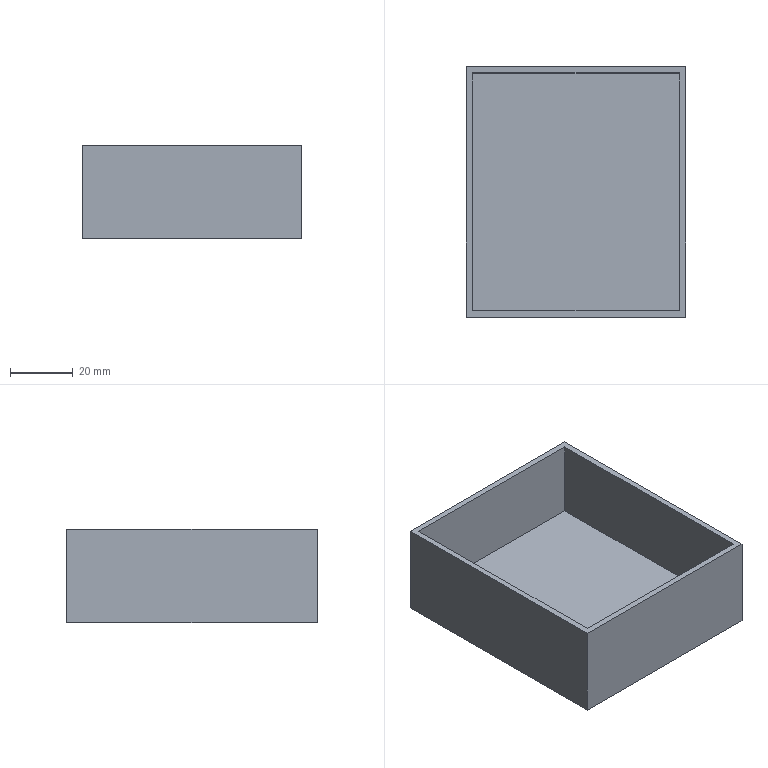Component | NX | REMOVABLE_STORAGE_1 | 1 solid | 11 faces | box 70 x 80 x 30 mm | volume 42600 mm3 | plane 11
STEP:
#1=CARTESIAN_POINT('',(0.,0.,0.));
#2=DIRECTION('',(0.,0.,1.));
#3=DIRECTION('',(1.,0.,0.));
#4=AXIS2_PLACEMENT_3D('',#1,#2,#3);
#5=CARTESIAN_POINT('',(145.,12.,35.));
#6=VERTEX_POINT('',#5);
#7=CARTESIAN_POINT('',(211.,12.,35.));
#8=VERTEX_POINT('',#7);
#9=CARTESIAN_POINT('',(145.,12.,35.));
#10=DIRECTION('',(1.,0.,0.));
#11=VECTOR('',#10,1.);
#12=LINE('',#9,#11);
#13=CARTESIAN_POINT('',(145.,12.,60.));
#14=DIRECTION('',(-0.,1.,0.));
#15=DIRECTION('',(-1.,-0.,0.));
#16=AXIS2_PLACEMENT_3D('',#13,#14,#15);
#17=PLANE('',#16);
#18=CARTESIAN_POINT('',(0.,-25.));
#19=DIRECTION('',(-1.,0.));
#20=VECTOR('',#19,1.);
#21=LINE('',#18,#20);
#22=(GEOMETRIC_REPRESENTATION_CONTEXT(2)PARAMETRIC_REPRESENTATION_CONTEXT()REPRESENTATION_CONTEXT('',''));
#23=DEFINITIONAL_REPRESENTATION('',(#21),#22);
#24=PCURVE('',#17,#23);
#25=CARTESIAN_POINT('',(143.,10.,35.));
#26=DIRECTION('',(0.,0.,1.));
#27=DIRECTION('',(1.,0.,0.));
#28=AXIS2_PLACEMENT_3D('',#25,#26,#27);
#29=PLANE('',#28);
#30=CARTESIAN_POINT('',(2.,2.));
#31=DIRECTION('',(1.,0.));
#32=VECTOR('',#31,1.);
#33=LINE('',#30,#32);
#34=(GEOMETRIC_REPRESENTATION_CONTEXT(2)PARAMETRIC_REPRESENTATION_CONTEXT()REPRESENTATION_CONTEXT('',''));
#35=DEFINITIONAL_REPRESENTATION('',(#33),#34);
#36=PCURVE('',#29,#35);
#37=SURFACE_CURVE('',#12,(#24,#36),.PCURVE_S1.);
#38=EDGE_CURVE('',#6,#8,#37,.T.);
#39=ORIENTED_EDGE('',*,*,#38,.F.);
#40=CARTESIAN_POINT('',(145.,12.,60.));
#41=VERTEX_POINT('',#40);
#42=CARTESIAN_POINT('',(145.,12.,60.));
#43=DIRECTION('',(0.,0.,-1.));
#44=VECTOR('',#43,1.);
#45=LINE('',#42,#44);
#46=CARTESIAN_POINT('',(0.,0.));
#47=DIRECTION('',(0.,-1.));
#48=VECTOR('',#47,1.);
#49=LINE('',#46,#48);
#50=(GEOMETRIC_REPRESENTATION_CONTEXT(2)PARAMETRIC_REPRESENTATION_CONTEXT()REPRESENTATION_CONTEXT('',''));
#51=DEFINITIONAL_REPRESENTATION('',(#49),#50);
#52=PCURVE('',#17,#51);
#53=CARTESIAN_POINT('',(145.,88.,60.));
#54=DIRECTION('',(1.,0.,0.));
#55=DIRECTION('',(-0.,1.,0.));
#56=AXIS2_PLACEMENT_3D('',#53,#54,#55);
#57=PLANE('',#56);
#58=CARTESIAN_POINT('',(-76.,0.));
#59=DIRECTION('',(0.,-1.));
#60=VECTOR('',#59,1.);
#61=LINE('',#58,#60);
#62=(GEOMETRIC_REPRESENTATION_CONTEXT(2)PARAMETRIC_REPRESENTATION_CONTEXT()REPRESENTATION_CONTEXT('',''));
#63=DEFINITIONAL_REPRESENTATION('',(#61),#62);
#64=PCURVE('',#57,#63);
#65=SURFACE_CURVE('',#45,(#52,#64),.PCURVE_S1.);
#66=EDGE_CURVE('',#41,#6,#65,.T.);
#67=ORIENTED_EDGE('',*,*,#66,.F.);
#68=CARTESIAN_POINT('',(211.,12.,60.));
#69=VERTEX_POINT('',#68);
#70=CARTESIAN_POINT('',(145.,12.,60.));
#71=DIRECTION('',(1.,0.,0.));
#72=VECTOR('',#71,1.);
#73=LINE('',#70,#72);
#74=CARTESIAN_POINT('',(0.,0.));
#75=DIRECTION('',(-1.,0.));
#76=VECTOR('',#75,1.);
#77=LINE('',#74,#76);
#78=(GEOMETRIC_REPRESENTATION_CONTEXT(2)PARAMETRIC_REPRESENTATION_CONTEXT()REPRESENTATION_CONTEXT('',''));
#79=DEFINITIONAL_REPRESENTATION('',(#77),#78);
#80=PCURVE('',#17,#79);
#81=CARTESIAN_POINT('',(143.,10.,60.));
#82=DIRECTION('',(0.,0.,-1.));
#83=DIRECTION('',(-1.,0.,0.));
#84=AXIS2_PLACEMENT_3D('',#81,#82,#83);
#85=PLANE('',#84);
#86=CARTESIAN_POINT('',(-2.,2.));
#87=DIRECTION('',(-1.,0.));
#88=VECTOR('',#87,1.);
#89=LINE('',#86,#88);
#90=(GEOMETRIC_REPRESENTATION_CONTEXT(2)PARAMETRIC_REPRESENTATION_CONTEXT()REPRESENTATION_CONTEXT('',''));
#91=DEFINITIONAL_REPRESENTATION('',(#89),#90);
#92=PCURVE('',#85,#91);
#93=SURFACE_CURVE('',#73,(#80,#92),.PCURVE_S1.);
#94=EDGE_CURVE('',#41,#69,#93,.T.);
#95=ORIENTED_EDGE('',*,*,#94,.T.);
#96=CARTESIAN_POINT('',(211.,12.,60.));
#97=DIRECTION('',(0.,0.,-1.));
#98=VECTOR('',#97,1.);
#99=LINE('',#96,#98);
#100=CARTESIAN_POINT('',(-66.,0.));
#101=DIRECTION('',(0.,-1.));
#102=VECTOR('',#101,1.);
#103=LINE('',#100,#102);
#104=(GEOMETRIC_REPRESENTATION_CONTEXT(2)PARAMETRIC_REPRESENTATION_CONTEXT()REPRESENTATION_CONTEXT('',''));
#105=DEFINITIONAL_REPRESENTATION('',(#103),#104);
#106=PCURVE('',#17,#105);
#107=CARTESIAN_POINT('',(211.,12.,60.));
#108=DIRECTION('',(-1.,0.,0.));
#109=DIRECTION('',(-0.,-1.,0.));
#110=AXIS2_PLACEMENT_3D('',#107,#108,#109);
#111=PLANE('',#110);
#112=CARTESIAN_POINT('',(0.,0.));
#113=DIRECTION('',(0.,-1.));
#114=VECTOR('',#113,1.);
#115=LINE('',#112,#114);
#116=(GEOMETRIC_REPRESENTATION_CONTEXT(2)PARAMETRIC_REPRESENTATION_CONTEXT()REPRESENTATION_CONTEXT('',''));
#117=DEFINITIONAL_REPRESENTATION('',(#115),#116);
#118=PCURVE('',#111,#117);
#119=SURFACE_CURVE('',#99,(#106,#118),.PCURVE_S1.);
#120=EDGE_CURVE('',#69,#8,#119,.T.);
#121=ORIENTED_EDGE('',*,*,#120,.T.);
#122=EDGE_LOOP('',(#39,#67,#95,#121));
#123=FACE_BOUND('',#122,.T.);
#124=ADVANCED_FACE('',(#123),#17,.T.);
#125=CARTESIAN_POINT('',(211.,88.,35.));
#126=VERTEX_POINT('',#125);
#127=CARTESIAN_POINT('',(211.,12.,35.));
#128=DIRECTION('',(0.,1.,0.));
#129=VECTOR('',#128,1.);
#130=LINE('',#127,#129);
#131=CARTESIAN_POINT('',(0.,-25.));
#132=DIRECTION('',(-1.,0.));
#133=VECTOR('',#132,1.);
#134=LINE('',#131,#133);
#135=(GEOMETRIC_REPRESENTATION_CONTEXT(2)PARAMETRIC_REPRESENTATION_CONTEXT()REPRESENTATION_CONTEXT('',''));
#136=DEFINITIONAL_REPRESENTATION('',(#134),#135);
#137=PCURVE('',#111,#136);
#138=CARTESIAN_POINT('',(68.,2.));
#139=DIRECTION('',(0.,1.));
#140=VECTOR('',#139,1.);
#141=LINE('',#138,#140);
#142=(GEOMETRIC_REPRESENTATION_CONTEXT(2)PARAMETRIC_REPRESENTATION_CONTEXT()REPRESENTATION_CONTEXT('',''));
#143=DEFINITIONAL_REPRESENTATION('',(#141),#142);
#144=PCURVE('',#29,#143);
#145=SURFACE_CURVE('',#130,(#137,#144),.PCURVE_S1.);
#146=EDGE_CURVE('',#8,#126,#145,.T.);
#147=ORIENTED_EDGE('',*,*,#146,.F.);
#148=ORIENTED_EDGE('',*,*,#120,.F.);
#149=CARTESIAN_POINT('',(211.,88.,60.));
#150=VERTEX_POINT('',#149);
#151=CARTESIAN_POINT('',(211.,12.,60.));
#152=DIRECTION('',(0.,1.,0.));
#153=VECTOR('',#152,1.);
#154=LINE('',#151,#153);
#155=CARTESIAN_POINT('',(0.,0.));
#156=DIRECTION('',(-1.,0.));
#157=VECTOR('',#156,1.);
#158=LINE('',#155,#157);
#159=(GEOMETRIC_REPRESENTATION_CONTEXT(2)PARAMETRIC_REPRESENTATION_CONTEXT()REPRESENTATION_CONTEXT('',''));
#160=DEFINITIONAL_REPRESENTATION('',(#158),#159);
#161=PCURVE('',#111,#160);
#162=CARTESIAN_POINT('',(-68.,2.));
#163=DIRECTION('',(-0.,1.));
#164=VECTOR('',#163,1.);
#165=LINE('',#162,#164);
#166=(GEOMETRIC_REPRESENTATION_CONTEXT(2)PARAMETRIC_REPRESENTATION_CONTEXT()REPRESENTATION_CONTEXT('',''));
#167=DEFINITIONAL_REPRESENTATION('',(#165),#166);
#168=PCURVE('',#85,#167);
#169=SURFACE_CURVE('',#154,(#161,#168),.PCURVE_S1.);
#170=EDGE_CURVE('',#69,#150,#169,.T.);
#171=ORIENTED_EDGE('',*,*,#170,.T.);
#172=CARTESIAN_POINT('',(211.,88.,60.));
#173=DIRECTION('',(0.,0.,-1.));
#174=VECTOR('',#173,1.);
#175=LINE('',#172,#174);
#176=CARTESIAN_POINT('',(-76.,0.));
#177=DIRECTION('',(0.,-1.));
#178=VECTOR('',#177,1.);
#179=LINE('',#176,#178);
#180=(GEOMETRIC_REPRESENTATION_CONTEXT(2)PARAMETRIC_REPRESENTATION_CONTEXT()REPRESENTATION_CONTEXT('',''));
#181=DEFINITIONAL_REPRESENTATION('',(#179),#180);
#182=PCURVE('',#111,#181);
#183=CARTESIAN_POINT('',(211.,88.,60.));
#184=DIRECTION('',(-0.,-1.,0.));
#185=DIRECTION('',(1.,-0.,0.));
#186=AXIS2_PLACEMENT_3D('',#183,#184,#185);
#187=PLANE('',#186);
#188=CARTESIAN_POINT('',(0.,0.));
#189=DIRECTION('',(0.,-1.));
#190=VECTOR('',#189,1.);
#191=LINE('',#188,#190);
#192=(GEOMETRIC_REPRESENTATION_CONTEXT(2)PARAMETRIC_REPRESENTATION_CONTEXT()REPRESENTATION_CONTEXT('',''));
#193=DEFINITIONAL_REPRESENTATION('',(#191),#192);
#194=PCURVE('',#187,#193);
#195=SURFACE_CURVE('',#175,(#182,#194),.PCURVE_S1.);
#196=EDGE_CURVE('',#150,#126,#195,.T.);
#197=ORIENTED_EDGE('',*,*,#196,.T.);
#198=EDGE_LOOP('',(#147,#148,#171,#197));
#199=FACE_BOUND('',#198,.T.);
#200=ADVANCED_FACE('',(#199),#111,.T.);
#201=CARTESIAN_POINT('',(145.,88.,35.));
#202=VERTEX_POINT('',#201);
#203=CARTESIAN_POINT('',(211.,88.,35.));
#204=DIRECTION('',(-1.,0.,0.));
#205=VECTOR('',#204,1.);
#206=LINE('',#203,#205);
#207=CARTESIAN_POINT('',(0.,-25.));
#208=DIRECTION('',(-1.,0.));
#209=VECTOR('',#208,1.);
#210=LINE('',#207,#209);
#211=(GEOMETRIC_REPRESENTATION_CONTEXT(2)PARAMETRIC_REPRESENTATION_CONTEXT()REPRESENTATION_CONTEXT('',''));
#212=DEFINITIONAL_REPRESENTATION('',(#210),#211);
#213=PCURVE('',#187,#212);
#214=CARTESIAN_POINT('',(68.,78.));
#215=DIRECTION('',(-1.,0.));
#216=VECTOR('',#215,1.);
#217=LINE('',#214,#216);
#218=(GEOMETRIC_REPRESENTATION_CONTEXT(2)PARAMETRIC_REPRESENTATION_CONTEXT()REPRESENTATION_CONTEXT('',''));
#219=DEFINITIONAL_REPRESENTATION('',(#217),#218);
#220=PCURVE('',#29,#219);
#221=SURFACE_CURVE('',#206,(#213,#220),.PCURVE_S1.);
#222=EDGE_CURVE('',#126,#202,#221,.T.);
#223=ORIENTED_EDGE('',*,*,#222,.F.);
#224=ORIENTED_EDGE('',*,*,#196,.F.);
#225=CARTESIAN_POINT('',(145.,88.,60.));
#226=VERTEX_POINT('',#225);
#227=CARTESIAN_POINT('',(211.,88.,60.));
#228=DIRECTION('',(-1.,0.,0.));
#229=VECTOR('',#228,1.);
#230=LINE('',#227,#229);
#231=CARTESIAN_POINT('',(0.,0.));
#232=DIRECTION('',(-1.,0.));
#233=VECTOR('',#232,1.);
#234=LINE('',#231,#233);
#235=(GEOMETRIC_REPRESENTATION_CONTEXT(2)PARAMETRIC_REPRESENTATION_CONTEXT()REPRESENTATION_CONTEXT('',''));
#236=DEFINITIONAL_REPRESENTATION('',(#234),#235);
#237=PCURVE('',#187,#236);
#238=CARTESIAN_POINT('',(-68.,78.));
#239=DIRECTION('',(1.,0.));
#240=VECTOR('',#239,1.);
#241=LINE('',#238,#240);
#242=(GEOMETRIC_REPRESENTATION_CONTEXT(2)PARAMETRIC_REPRESENTATION_CONTEXT()REPRESENTATION_CONTEXT('',''));
#243=DEFINITIONAL_REPRESENTATION('',(#241),#242);
#244=PCURVE('',#85,#243);
#245=SURFACE_CURVE('',#230,(#237,#244),.PCURVE_S1.);
#246=EDGE_CURVE('',#150,#226,#245,.T.);
#247=ORIENTED_EDGE('',*,*,#246,.T.);
#248=CARTESIAN_POINT('',(145.,88.,60.));
#249=DIRECTION('',(0.,0.,-1.));
#250=VECTOR('',#249,1.);
#251=LINE('',#248,#250);
#252=CARTESIAN_POINT('',(-66.,0.));
#253=DIRECTION('',(0.,-1.));
#254=VECTOR('',#253,1.);
#255=LINE('',#252,#254);
#256=(GEOMETRIC_REPRESENTATION_CONTEXT(2)PARAMETRIC_REPRESENTATION_CONTEXT()REPRESENTATION_CONTEXT('',''));
#257=DEFINITIONAL_REPRESENTATION('',(#255),#256);
#258=PCURVE('',#187,#257);
#259=CARTESIAN_POINT('',(0.,0.));
#260=DIRECTION('',(0.,-1.));
#261=VECTOR('',#260,1.);
#262=LINE('',#259,#261);
#263=(GEOMETRIC_REPRESENTATION_CONTEXT(2)PARAMETRIC_REPRESENTATION_CONTEXT()REPRESENTATION_CONTEXT('',''));
#264=DEFINITIONAL_REPRESENTATION('',(#262),#263);
#265=PCURVE('',#57,#264);
#266=SURFACE_CURVE('',#251,(#258,#265),.PCURVE_S1.);
#267=EDGE_CURVE('',#226,#202,#266,.T.);
#268=ORIENTED_EDGE('',*,*,#267,.T.);
#269=EDGE_LOOP('',(#223,#224,#247,#268));
#270=FACE_BOUND('',#269,.T.);
#271=ADVANCED_FACE('',(#270),#187,.T.);
#272=CARTESIAN_POINT('',(143.,90.,30.));
#273=VERTEX_POINT('',#272);
#274=CARTESIAN_POINT('',(213.,90.,30.));
#275=VERTEX_POINT('',#274);
#276=CARTESIAN_POINT('',(143.,90.,30.));
#277=DIRECTION('',(1.,0.,0.));
#278=VECTOR('',#277,1.);
#279=LINE('',#276,#278);
#280=CARTESIAN_POINT('',(143.,90.,60.));
#281=DIRECTION('',(0.,1.,0.));
#282=DIRECTION('',(0.,0.,1.));
#283=AXIS2_PLACEMENT_3D('',#280,#281,#282);
#284=PLANE('',#283);
#285=CARTESIAN_POINT('',(-30.,0.));
#286=DIRECTION('',(0.,1.));
#287=VECTOR('',#286,1.);
#288=LINE('',#285,#287);
#289=(GEOMETRIC_REPRESENTATION_CONTEXT(2)PARAMETRIC_REPRESENTATION_CONTEXT()REPRESENTATION_CONTEXT('',''));
#290=DEFINITIONAL_REPRESENTATION('',(#288),#289);
#291=PCURVE('',#284,#290);
#292=CARTESIAN_POINT('',(143.,10.,30.));
#293=DIRECTION('',(0.,0.,-1.));
#294=DIRECTION('',(-1.,0.,0.));
#295=AXIS2_PLACEMENT_3D('',#292,#293,#294);
#296=PLANE('',#295);
#297=CARTESIAN_POINT('',(0.,80.));
#298=DIRECTION('',(-1.,0.));
#299=VECTOR('',#298,1.);
#300=LINE('',#297,#299);
#301=(GEOMETRIC_REPRESENTATION_CONTEXT(2)PARAMETRIC_REPRESENTATION_CONTEXT()REPRESENTATION_CONTEXT('',''));
#302=DEFINITIONAL_REPRESENTATION('',(#300),#301);
#303=PCURVE('',#296,#302);
#304=SURFACE_CURVE('',#279,(#291,#303),.PCURVE_S1.);
#305=EDGE_CURVE('',#273,#275,#304,.T.);
#306=ORIENTED_EDGE('',*,*,#305,.F.);
#307=CARTESIAN_POINT('',(143.,90.,60.));
#308=VERTEX_POINT('',#307);
#309=CARTESIAN_POINT('',(143.,90.,60.));
#310=DIRECTION('',(0.,0.,-1.));
#311=VECTOR('',#310,1.);
#312=LINE('',#309,#311);
#313=CARTESIAN_POINT('',(0.,0.));
#314=DIRECTION('',(-1.,0.));
#315=VECTOR('',#314,1.);
#316=LINE('',#313,#315);
#317=(GEOMETRIC_REPRESENTATION_CONTEXT(2)PARAMETRIC_REPRESENTATION_CONTEXT()REPRESENTATION_CONTEXT('',''));
#318=DEFINITIONAL_REPRESENTATION('',(#316),#317);
#319=PCURVE('',#284,#318);
#320=CARTESIAN_POINT('',(143.,10.,60.));
#321=DIRECTION('',(-1.,0.,0.));
#322=DIRECTION('',(0.,0.,1.));
#323=AXIS2_PLACEMENT_3D('',#320,#321,#322);
#324=PLANE('',#323);
#325=CARTESIAN_POINT('',(0.,80.));
#326=DIRECTION('',(-1.,0.));
#327=VECTOR('',#326,1.);
#328=LINE('',#325,#327);
#329=(GEOMETRIC_REPRESENTATION_CONTEXT(2)PARAMETRIC_REPRESENTATION_CONTEXT()REPRESENTATION_CONTEXT('',''));
#330=DEFINITIONAL_REPRESENTATION('',(#328),#329);
#331=PCURVE('',#324,#330);
#332=SURFACE_CURVE('',#312,(#319,#331),.PCURVE_S1.);
#333=EDGE_CURVE('',#308,#273,#332,.T.);
#334=ORIENTED_EDGE('',*,*,#333,.F.);
#335=CARTESIAN_POINT('',(213.,90.,60.));
#336=VERTEX_POINT('',#335);
#337=CARTESIAN_POINT('',(143.,90.,60.));
#338=DIRECTION('',(1.,0.,0.));
#339=VECTOR('',#338,1.);
#340=LINE('',#337,#339);
#341=CARTESIAN_POINT('',(0.,0.));
#342=DIRECTION('',(0.,1.));
#343=VECTOR('',#342,1.);
#344=LINE('',#341,#343);
#345=(GEOMETRIC_REPRESENTATION_CONTEXT(2)PARAMETRIC_REPRESENTATION_CONTEXT()REPRESENTATION_CONTEXT('',''));
#346=DEFINITIONAL_REPRESENTATION('',(#344),#345);
#347=PCURVE('',#284,#346);
#348=CARTESIAN_POINT('',(0.,80.));
#349=DIRECTION('',(-1.,0.));
#350=VECTOR('',#349,1.);
#351=LINE('',#348,#350);
#352=(GEOMETRIC_REPRESENTATION_CONTEXT(2)PARAMETRIC_REPRESENTATION_CONTEXT()REPRESENTATION_CONTEXT('',''));
#353=DEFINITIONAL_REPRESENTATION('',(#351),#352);
#354=PCURVE('',#85,#353);
#355=SURFACE_CURVE('',#340,(#347,#354),.PCURVE_S1.);
#356=EDGE_CURVE('',#308,#336,#355,.T.);
#357=ORIENTED_EDGE('',*,*,#356,.T.);
#358=CARTESIAN_POINT('',(213.,90.,60.));
#359=DIRECTION('',(0.,0.,-1.));
#360=VECTOR('',#359,1.);
#361=LINE('',#358,#360);
#362=CARTESIAN_POINT('',(0.,70.));
#363=DIRECTION('',(-1.,0.));
#364=VECTOR('',#363,1.);
#365=LINE('',#362,#364);
#366=(GEOMETRIC_REPRESENTATION_CONTEXT(2)PARAMETRIC_REPRESENTATION_CONTEXT()REPRESENTATION_CONTEXT('',''));
#367=DEFINITIONAL_REPRESENTATION('',(#365),#366);
#368=PCURVE('',#284,#367);
#369=CARTESIAN_POINT('',(213.,90.,60.));
#370=DIRECTION('',(1.,0.,0.));
#371=DIRECTION('',(0.,0.,-1.));
#372=AXIS2_PLACEMENT_3D('',#369,#370,#371);
#373=PLANE('',#372);
#374=CARTESIAN_POINT('',(0.,0.));
#375=DIRECTION('',(1.,0.));
#376=VECTOR('',#375,1.);
#377=LINE('',#374,#376);
#378=(GEOMETRIC_REPRESENTATION_CONTEXT(2)PARAMETRIC_REPRESENTATION_CONTEXT()REPRESENTATION_CONTEXT('',''));
#379=DEFINITIONAL_REPRESENTATION('',(#377),#378);
#380=PCURVE('',#373,#379);
#381=SURFACE_CURVE('',#361,(#368,#380),.PCURVE_S1.);
#382=EDGE_CURVE('',#336,#275,#381,.T.);
#383=ORIENTED_EDGE('',*,*,#382,.T.);
#384=EDGE_LOOP('',(#306,#334,#357,#383));
#385=FACE_BOUND('',#384,.T.);
#386=ADVANCED_FACE('',(#385),#284,.T.);
#387=CARTESIAN_POINT('',(213.,10.,30.));
#388=VERTEX_POINT('',#387);
#389=CARTESIAN_POINT('',(213.,90.,30.));
#390=DIRECTION('',(0.,-1.,0.));
#391=VECTOR('',#390,1.);
#392=LINE('',#389,#391);
#393=CARTESIAN_POINT('',(30.,0.));
#394=DIRECTION('',(0.,-1.));
#395=VECTOR('',#394,1.);
#396=LINE('',#393,#395);
#397=(GEOMETRIC_REPRESENTATION_CONTEXT(2)PARAMETRIC_REPRESENTATION_CONTEXT()REPRESENTATION_CONTEXT('',''));
#398=DEFINITIONAL_REPRESENTATION('',(#396),#397);
#399=PCURVE('',#373,#398);
#400=CARTESIAN_POINT('',(-70.,80.));
#401=DIRECTION('',(0.,-1.));
#402=VECTOR('',#401,1.);
#403=LINE('',#400,#402);
#404=(GEOMETRIC_REPRESENTATION_CONTEXT(2)PARAMETRIC_REPRESENTATION_CONTEXT()REPRESENTATION_CONTEXT('',''));
#405=DEFINITIONAL_REPRESENTATION('',(#403),#404);
#406=PCURVE('',#296,#405);
#407=SURFACE_CURVE('',#392,(#399,#406),.PCURVE_S1.);
#408=EDGE_CURVE('',#275,#388,#407,.T.);
#409=ORIENTED_EDGE('',*,*,#408,.F.);
#410=ORIENTED_EDGE('',*,*,#382,.F.);
#411=CARTESIAN_POINT('',(213.,10.,60.));
#412=VERTEX_POINT('',#411);
#413=CARTESIAN_POINT('',(213.,90.,60.));
#414=DIRECTION('',(0.,-1.,0.));
#415=VECTOR('',#414,1.);
#416=LINE('',#413,#415);
#417=CARTESIAN_POINT('',(0.,0.));
#418=DIRECTION('',(0.,-1.));
#419=VECTOR('',#418,1.);
#420=LINE('',#417,#419);
#421=(GEOMETRIC_REPRESENTATION_CONTEXT(2)PARAMETRIC_REPRESENTATION_CONTEXT()REPRESENTATION_CONTEXT('',''));
#422=DEFINITIONAL_REPRESENTATION('',(#420),#421);
#423=PCURVE('',#373,#422);
#424=CARTESIAN_POINT('',(-70.,80.));
#425=DIRECTION('',(0.,-1.));
#426=VECTOR('',#425,1.);
#427=LINE('',#424,#426);
#428=(GEOMETRIC_REPRESENTATION_CONTEXT(2)PARAMETRIC_REPRESENTATION_CONTEXT()REPRESENTATION_CONTEXT('',''));
#429=DEFINITIONAL_REPRESENTATION('',(#427),#428);
#430=PCURVE('',#85,#429);
#431=SURFACE_CURVE('',#416,(#423,#430),.PCURVE_S1.);
#432=EDGE_CURVE('',#336,#412,#431,.T.);
#433=ORIENTED_EDGE('',*,*,#432,.T.);
#434=CARTESIAN_POINT('',(213.,10.,60.));
#435=DIRECTION('',(0.,0.,-1.));
#436=VECTOR('',#435,1.);
#437=LINE('',#434,#436);
#438=CARTESIAN_POINT('',(0.,-80.));
#439=DIRECTION('',(1.,0.));
#440=VECTOR('',#439,1.);
#441=LINE('',#438,#440);
#442=(GEOMETRIC_REPRESENTATION_CONTEXT(2)PARAMETRIC_REPRESENTATION_CONTEXT()REPRESENTATION_CONTEXT('',''));
#443=DEFINITIONAL_REPRESENTATION('',(#441),#442);
#444=PCURVE('',#373,#443);
#445=CARTESIAN_POINT('',(213.,10.,60.));
#446=DIRECTION('',(0.,-1.,0.));
#447=DIRECTION('',(0.,0.,-1.));
#448=AXIS2_PLACEMENT_3D('',#445,#446,#447);
#449=PLANE('',#448);
#450=CARTESIAN_POINT('',(0.,0.));
#451=DIRECTION('',(1.,0.));
#452=VECTOR('',#451,1.);
#453=LINE('',#450,#452);
#454=(GEOMETRIC_REPRESENTATION_CONTEXT(2)PARAMETRIC_REPRESENTATION_CONTEXT()REPRESENTATION_CONTEXT('',''));
#455=DEFINITIONAL_REPRESENTATION('',(#453),#454);
#456=PCURVE('',#449,#455);
#457=SURFACE_CURVE('',#437,(#444,#456),.PCURVE_S1.);
#458=EDGE_CURVE('',#412,#388,#457,.T.);
#459=ORIENTED_EDGE('',*,*,#458,.T.);
#460=EDGE_LOOP('',(#409,#410,#433,#459));
#461=FACE_BOUND('',#460,.T.);
#462=ADVANCED_FACE('',(#461),#373,.T.);
#463=CARTESIAN_POINT('',(143.,10.,30.));
#464=VERTEX_POINT('',#463);
#465=CARTESIAN_POINT('',(213.,10.,30.));
#466=DIRECTION('',(-1.,0.,0.));
#467=VECTOR('',#466,1.);
#468=LINE('',#465,#467);
#469=CARTESIAN_POINT('',(30.,0.));
#470=DIRECTION('',(0.,-1.));
#471=VECTOR('',#470,1.);
#472=LINE('',#469,#471);
#473=(GEOMETRIC_REPRESENTATION_CONTEXT(2)PARAMETRIC_REPRESENTATION_CONTEXT()REPRESENTATION_CONTEXT('',''));
#474=DEFINITIONAL_REPRESENTATION('',(#472),#473);
#475=PCURVE('',#449,#474);
#476=CARTESIAN_POINT('',(-70.,0.));
#477=DIRECTION('',(1.,0.));
#478=VECTOR('',#477,1.);
#479=LINE('',#476,#478);
#480=(GEOMETRIC_REPRESENTATION_CONTEXT(2)PARAMETRIC_REPRESENTATION_CONTEXT()REPRESENTATION_CONTEXT('',''));
#481=DEFINITIONAL_REPRESENTATION('',(#479),#480);
#482=PCURVE('',#296,#481);
#483=SURFACE_CURVE('',#468,(#475,#482),.PCURVE_S1.);
#484=EDGE_CURVE('',#388,#464,#483,.T.);
#485=ORIENTED_EDGE('',*,*,#484,.F.);
#486=ORIENTED_EDGE('',*,*,#458,.F.);
#487=CARTESIAN_POINT('',(143.,10.,60.));
#488=VERTEX_POINT('',#487);
#489=CARTESIAN_POINT('',(213.,10.,60.));
#490=DIRECTION('',(-1.,0.,0.));
#491=VECTOR('',#490,1.);
#492=LINE('',#489,#491);
#493=CARTESIAN_POINT('',(0.,0.));
#494=DIRECTION('',(0.,-1.));
#495=VECTOR('',#494,1.);
#496=LINE('',#493,#495);
#497=(GEOMETRIC_REPRESENTATION_CONTEXT(2)PARAMETRIC_REPRESENTATION_CONTEXT()REPRESENTATION_CONTEXT('',''));
#498=DEFINITIONAL_REPRESENTATION('',(#496),#497);
#499=PCURVE('',#449,#498);
#500=CARTESIAN_POINT('',(-70.,0.));
#501=DIRECTION('',(1.,0.));
#502=VECTOR('',#501,1.);
#503=LINE('',#500,#502);
#504=(GEOMETRIC_REPRESENTATION_CONTEXT(2)PARAMETRIC_REPRESENTATION_CONTEXT()REPRESENTATION_CONTEXT('',''));
#505=DEFINITIONAL_REPRESENTATION('',(#503),#504);
#506=PCURVE('',#85,#505);
#507=SURFACE_CURVE('',#492,(#499,#506),.PCURVE_S1.);
#508=EDGE_CURVE('',#412,#488,#507,.T.);
#509=ORIENTED_EDGE('',*,*,#508,.T.);
#510=CARTESIAN_POINT('',(143.,10.,60.));
#511=DIRECTION('',(0.,0.,-1.));
#512=VECTOR('',#511,1.);
#513=LINE('',#510,#512);
#514=CARTESIAN_POINT('',(0.,-70.));
#515=DIRECTION('',(1.,0.));
#516=VECTOR('',#515,1.);
#517=LINE('',#514,#516);
#518=(GEOMETRIC_REPRESENTATION_CONTEXT(2)PARAMETRIC_REPRESENTATION_CONTEXT()REPRESENTATION_CONTEXT('',''));
#519=DEFINITIONAL_REPRESENTATION('',(#517),#518);
#520=PCURVE('',#449,#519);
#521=CARTESIAN_POINT('',(0.,0.));
#522=DIRECTION('',(-1.,0.));
#523=VECTOR('',#522,1.);
#524=LINE('',#521,#523);
#525=(GEOMETRIC_REPRESENTATION_CONTEXT(2)PARAMETRIC_REPRESENTATION_CONTEXT()REPRESENTATION_CONTEXT('',''));
#526=DEFINITIONAL_REPRESENTATION('',(#524),#525);
#527=PCURVE('',#324,#526);
#528=SURFACE_CURVE('',#513,(#520,#527),.PCURVE_S1.);
#529=EDGE_CURVE('',#488,#464,#528,.T.);
#530=ORIENTED_EDGE('',*,*,#529,.T.);
#531=EDGE_LOOP('',(#485,#486,#509,#530));
#532=FACE_BOUND('',#531,.T.);
#533=ADVANCED_FACE('',(#532),#449,.T.);
#534=CARTESIAN_POINT('',(143.,10.,30.));
#535=DIRECTION('',(0.,1.,0.));
#536=VECTOR('',#535,1.);
#537=LINE('',#534,#536);
#538=CARTESIAN_POINT('',(-30.,0.));
#539=DIRECTION('',(0.,1.));
#540=VECTOR('',#539,1.);
#541=LINE('',#538,#540);
#542=(GEOMETRIC_REPRESENTATION_CONTEXT(2)PARAMETRIC_REPRESENTATION_CONTEXT()REPRESENTATION_CONTEXT('',''));
#543=DEFINITIONAL_REPRESENTATION('',(#541),#542);
#544=PCURVE('',#324,#543);
#545=CARTESIAN_POINT('',(0.,0.));
#546=DIRECTION('',(0.,1.));
#547=VECTOR('',#546,1.);
#548=LINE('',#545,#547);
#549=(GEOMETRIC_REPRESENTATION_CONTEXT(2)PARAMETRIC_REPRESENTATION_CONTEXT()REPRESENTATION_CONTEXT('',''));
#550=DEFINITIONAL_REPRESENTATION('',(#548),#549);
#551=PCURVE('',#296,#550);
#552=SURFACE_CURVE('',#537,(#544,#551),.PCURVE_S1.);
#553=EDGE_CURVE('',#464,#273,#552,.T.);
#554=ORIENTED_EDGE('',*,*,#553,.F.);
#555=ORIENTED_EDGE('',*,*,#529,.F.);
#556=CARTESIAN_POINT('',(143.,10.,60.));
#557=DIRECTION('',(0.,1.,0.));
#558=VECTOR('',#557,1.);
#559=LINE('',#556,#558);
#560=CARTESIAN_POINT('',(0.,0.));
#561=DIRECTION('',(0.,1.));
#562=VECTOR('',#561,1.);
#563=LINE('',#560,#562);
#564=(GEOMETRIC_REPRESENTATION_CONTEXT(2)PARAMETRIC_REPRESENTATION_CONTEXT()REPRESENTATION_CONTEXT('',''));
#565=DEFINITIONAL_REPRESENTATION('',(#563),#564);
#566=PCURVE('',#324,#565);
#567=CARTESIAN_POINT('',(0.,0.));
#568=DIRECTION('',(0.,1.));
#569=VECTOR('',#568,1.);
#570=LINE('',#567,#569);
#571=(GEOMETRIC_REPRESENTATION_CONTEXT(2)PARAMETRIC_REPRESENTATION_CONTEXT()REPRESENTATION_CONTEXT('',''));
#572=DEFINITIONAL_REPRESENTATION('',(#570),#571);
#573=PCURVE('',#85,#572);
#574=SURFACE_CURVE('',#559,(#566,#573),.PCURVE_S1.);
#575=EDGE_CURVE('',#488,#308,#574,.T.);
#576=ORIENTED_EDGE('',*,*,#575,.T.);
#577=ORIENTED_EDGE('',*,*,#333,.T.);
#578=EDGE_LOOP('',(#554,#555,#576,#577));
#579=FACE_BOUND('',#578,.T.);
#580=ADVANCED_FACE('',(#579),#324,.T.);
#581=CARTESIAN_POINT('',(145.,88.,35.));
#582=DIRECTION('',(0.,-1.,0.));
#583=VECTOR('',#582,1.);
#584=LINE('',#581,#583);
#585=CARTESIAN_POINT('',(0.,-25.));
#586=DIRECTION('',(-1.,0.));
#587=VECTOR('',#586,1.);
#588=LINE('',#585,#587);
#589=(GEOMETRIC_REPRESENTATION_CONTEXT(2)PARAMETRIC_REPRESENTATION_CONTEXT()REPRESENTATION_CONTEXT('',''));
#590=DEFINITIONAL_REPRESENTATION('',(#588),#589);
#591=PCURVE('',#57,#590);
#592=CARTESIAN_POINT('',(2.,78.));
#593=DIRECTION('',(0.,-1.));
#594=VECTOR('',#593,1.);
#595=LINE('',#592,#594);
#596=(GEOMETRIC_REPRESENTATION_CONTEXT(2)PARAMETRIC_REPRESENTATION_CONTEXT()REPRESENTATION_CONTEXT('',''));
#597=DEFINITIONAL_REPRESENTATION('',(#595),#596);
#598=PCURVE('',#29,#597);
#599=SURFACE_CURVE('',#584,(#591,#598),.PCURVE_S1.);
#600=EDGE_CURVE('',#202,#6,#599,.T.);
#601=ORIENTED_EDGE('',*,*,#600,.F.);
#602=ORIENTED_EDGE('',*,*,#267,.F.);
#603=CARTESIAN_POINT('',(145.,88.,60.));
#604=DIRECTION('',(0.,-1.,0.));
#605=VECTOR('',#604,1.);
#606=LINE('',#603,#605);
#607=CARTESIAN_POINT('',(0.,0.));
#608=DIRECTION('',(-1.,0.));
#609=VECTOR('',#608,1.);
#610=LINE('',#607,#609);
#611=(GEOMETRIC_REPRESENTATION_CONTEXT(2)PARAMETRIC_REPRESENTATION_CONTEXT()REPRESENTATION_CONTEXT('',''));
#612=DEFINITIONAL_REPRESENTATION('',(#610),#611);
#613=PCURVE('',#57,#612);
#614=CARTESIAN_POINT('',(-2.,78.));
#615=DIRECTION('',(-0.,-1.));
#616=VECTOR('',#615,1.);
#617=LINE('',#614,#616);
#618=(GEOMETRIC_REPRESENTATION_CONTEXT(2)PARAMETRIC_REPRESENTATION_CONTEXT()REPRESENTATION_CONTEXT('',''));
#619=DEFINITIONAL_REPRESENTATION('',(#617),#618);
#620=PCURVE('',#85,#619);
#621=SURFACE_CURVE('',#606,(#613,#620),.PCURVE_S1.);
#622=EDGE_CURVE('',#226,#41,#621,.T.);
#623=ORIENTED_EDGE('',*,*,#622,.T.);
#624=ORIENTED_EDGE('',*,*,#66,.T.);
#625=EDGE_LOOP('',(#601,#602,#623,#624));
#626=FACE_BOUND('',#625,.T.);
#627=ADVANCED_FACE('',(#626),#57,.T.);
#628=ORIENTED_EDGE('',*,*,#356,.F.);
#629=ORIENTED_EDGE('',*,*,#575,.F.);
#630=ORIENTED_EDGE('',*,*,#508,.F.);
#631=ORIENTED_EDGE('',*,*,#432,.F.);
#632=EDGE_LOOP('',(#628,#629,#630,#631));
#633=FACE_BOUND('',#632,.T.);
#634=ORIENTED_EDGE('',*,*,#94,.F.);
#635=ORIENTED_EDGE('',*,*,#622,.F.);
#636=ORIENTED_EDGE('',*,*,#246,.F.);
#637=ORIENTED_EDGE('',*,*,#170,.F.);
#638=EDGE_LOOP('',(#634,#635,#636,#637));
#639=FACE_BOUND('',#638,.T.);
#640=ADVANCED_FACE('',(#633,#639),#85,.F.);
#641=ORIENTED_EDGE('',*,*,#305,.T.);
#642=ORIENTED_EDGE('',*,*,#408,.T.);
#643=ORIENTED_EDGE('',*,*,#484,.T.);
#644=ORIENTED_EDGE('',*,*,#553,.T.);
#645=EDGE_LOOP('',(#641,#642,#643,#644));
#646=FACE_BOUND('',#645,.T.);
#647=ADVANCED_FACE('',(#646),#296,.T.);
#648=ORIENTED_EDGE('',*,*,#600,.T.);
#649=ORIENTED_EDGE('',*,*,#38,.T.);
#650=ORIENTED_EDGE('',*,*,#146,.T.);
#651=ORIENTED_EDGE('',*,*,#222,.T.);
#652=EDGE_LOOP('',(#648,#649,#650,#651));
#653=FACE_BOUND('',#652,.T.);
#654=ADVANCED_FACE('',(#653),#29,.T.);
#655=CLOSED_SHELL('',(#124,#200,#271,#386,#462,#533,#580,#627,#640,#647,#654));
#656=MANIFOLD_SOLID_BREP('',#655);
#657=(LENGTH_UNIT()NAMED_UNIT(*)SI_UNIT(.MILLI.,.METRE.));
#658=UNCERTAINTY_MEASURE_WITH_UNIT(LENGTH_MEASURE(0.0000001),#657,'','');
#659=(NAMED_UNIT(*)PLANE_ANGLE_UNIT()SI_UNIT($,.RADIAN.));
#660=(NAMED_UNIT(*)SI_UNIT($,.STERADIAN.)SOLID_ANGLE_UNIT());
#661=(GEOMETRIC_REPRESENTATION_CONTEXT(3)GLOBAL_UNCERTAINTY_ASSIGNED_CONTEXT((#658))GLOBAL_UNIT_ASSIGNED_CONTEXT((#657,#659,#660))REPRESENTATION_CONTEXT('',''));
#662=ADVANCED_BREP_SHAPE_REPRESENTATION('',(#4,#656),#661);